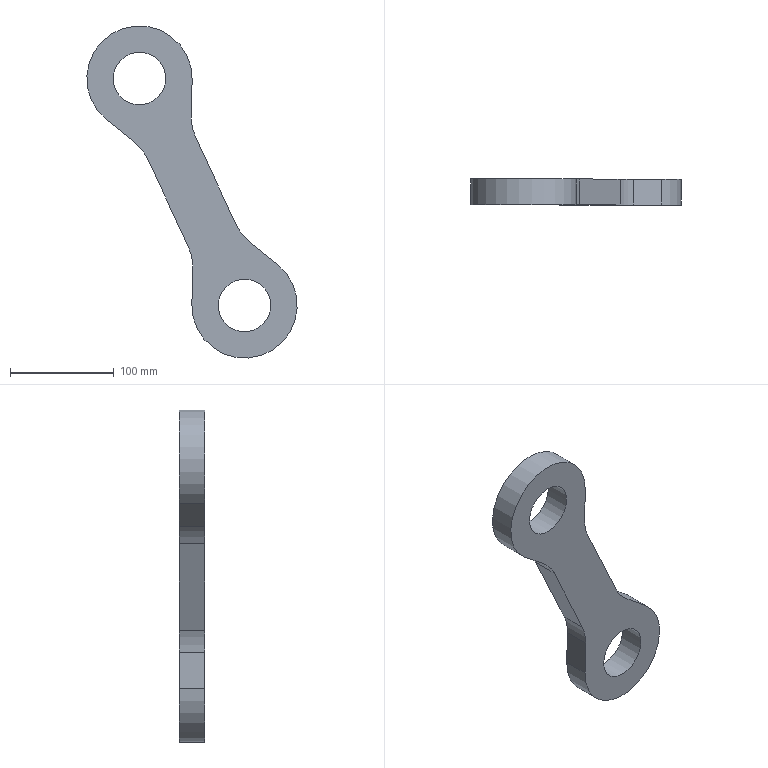Component | NX | CONNECTOR_1 | 1 solid | 16 faces | volume 503281 mm3 | plane 8 | cylinder 8 | commonest cylinder face diameters 94 x4 101.6 x2 50.8 x2